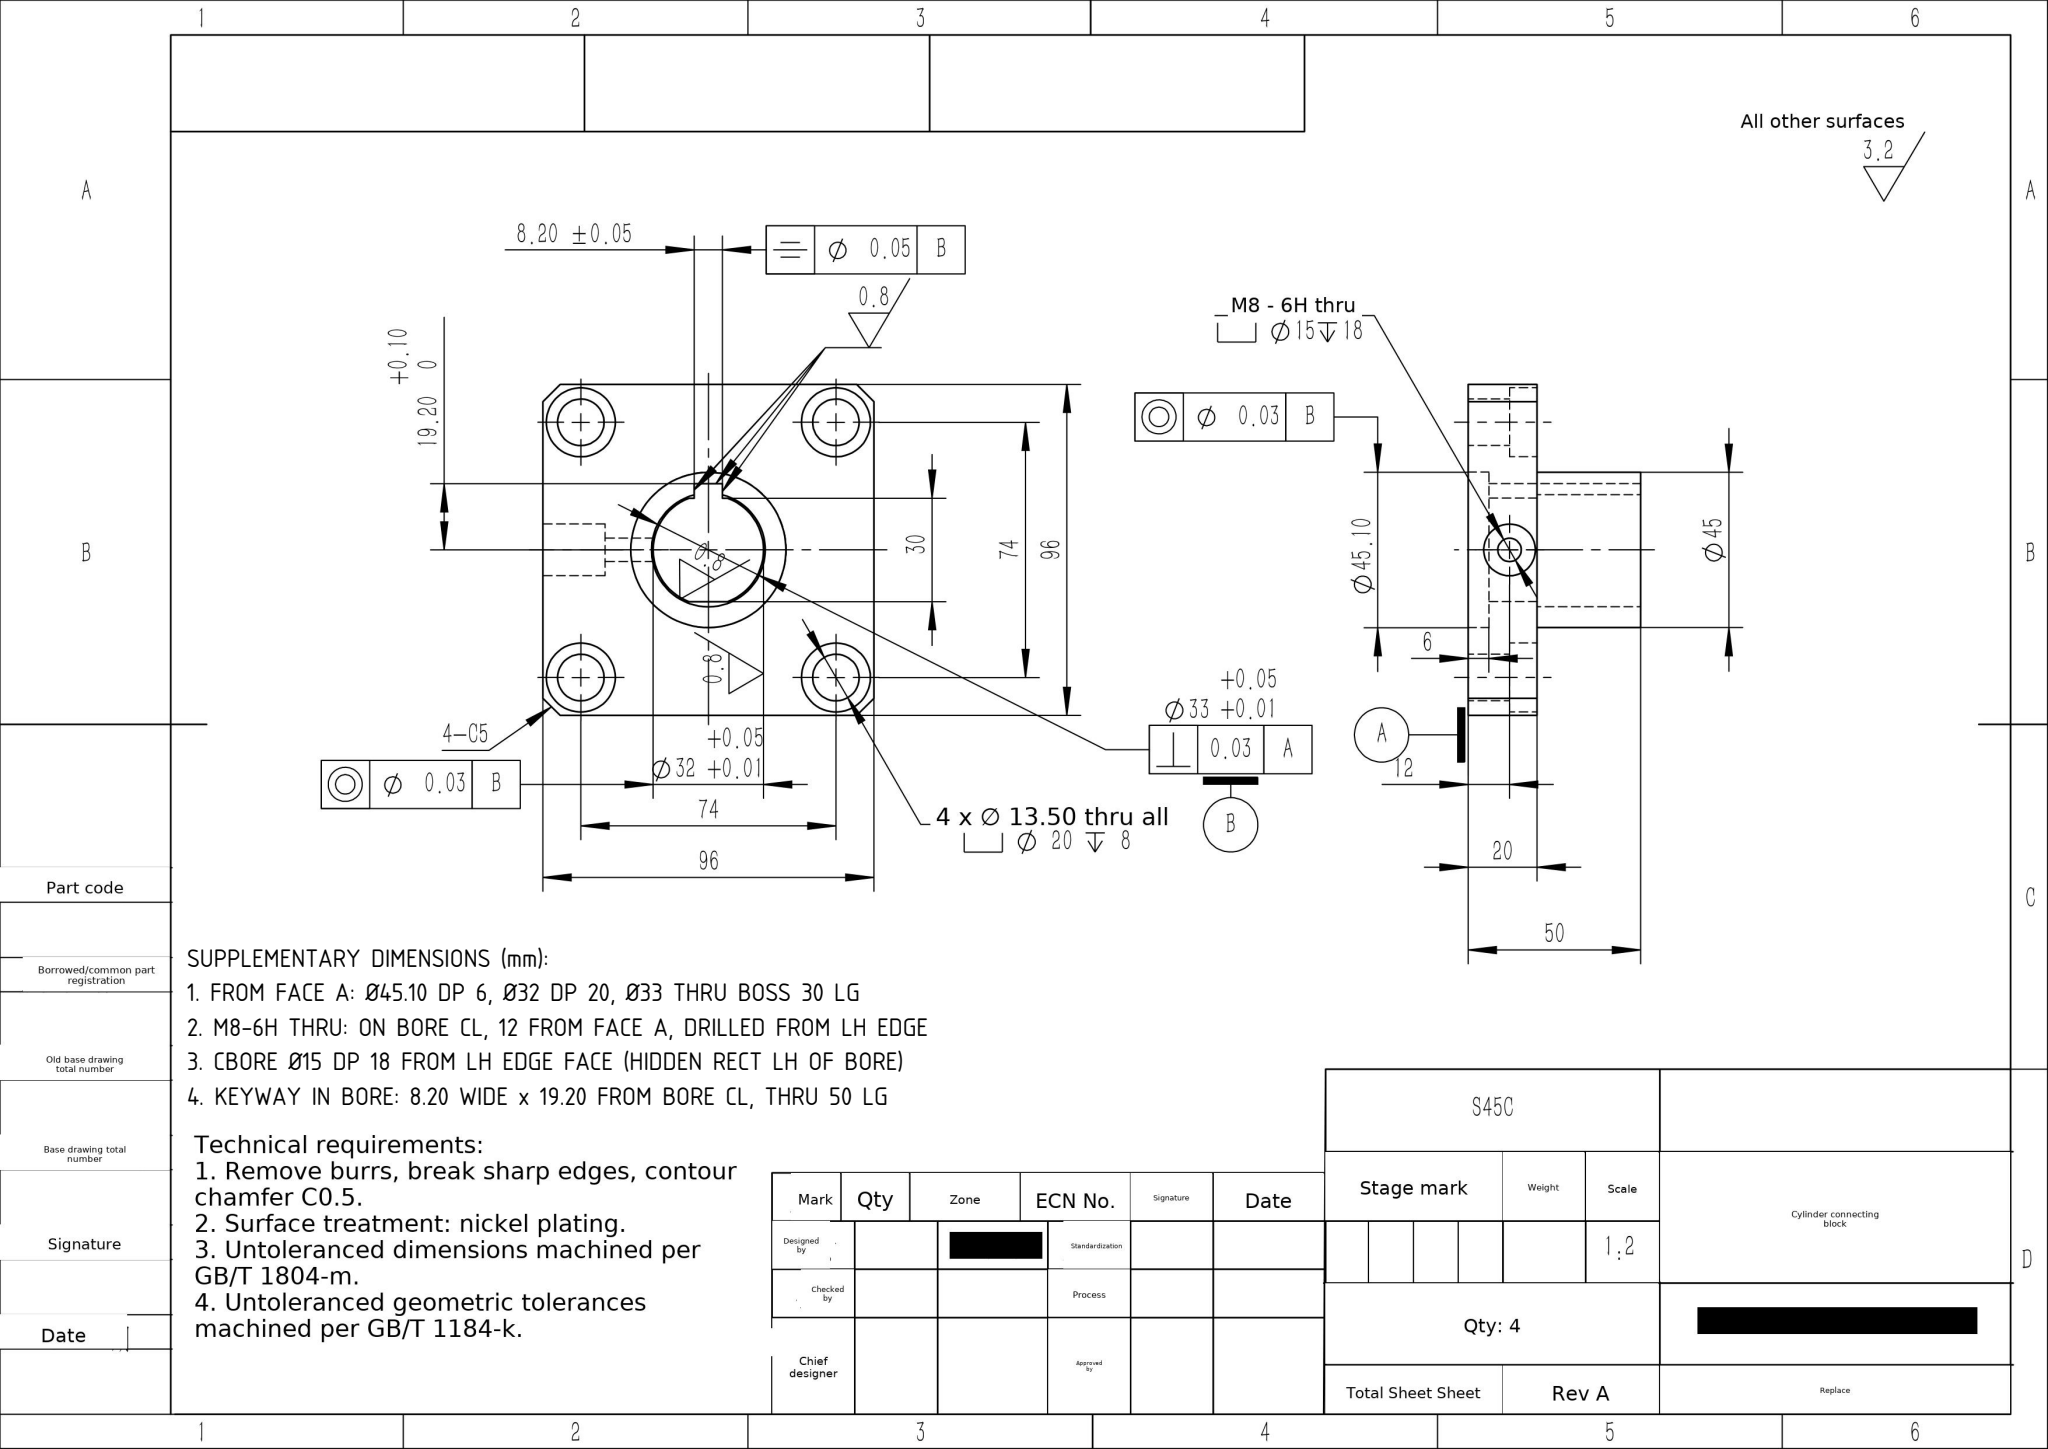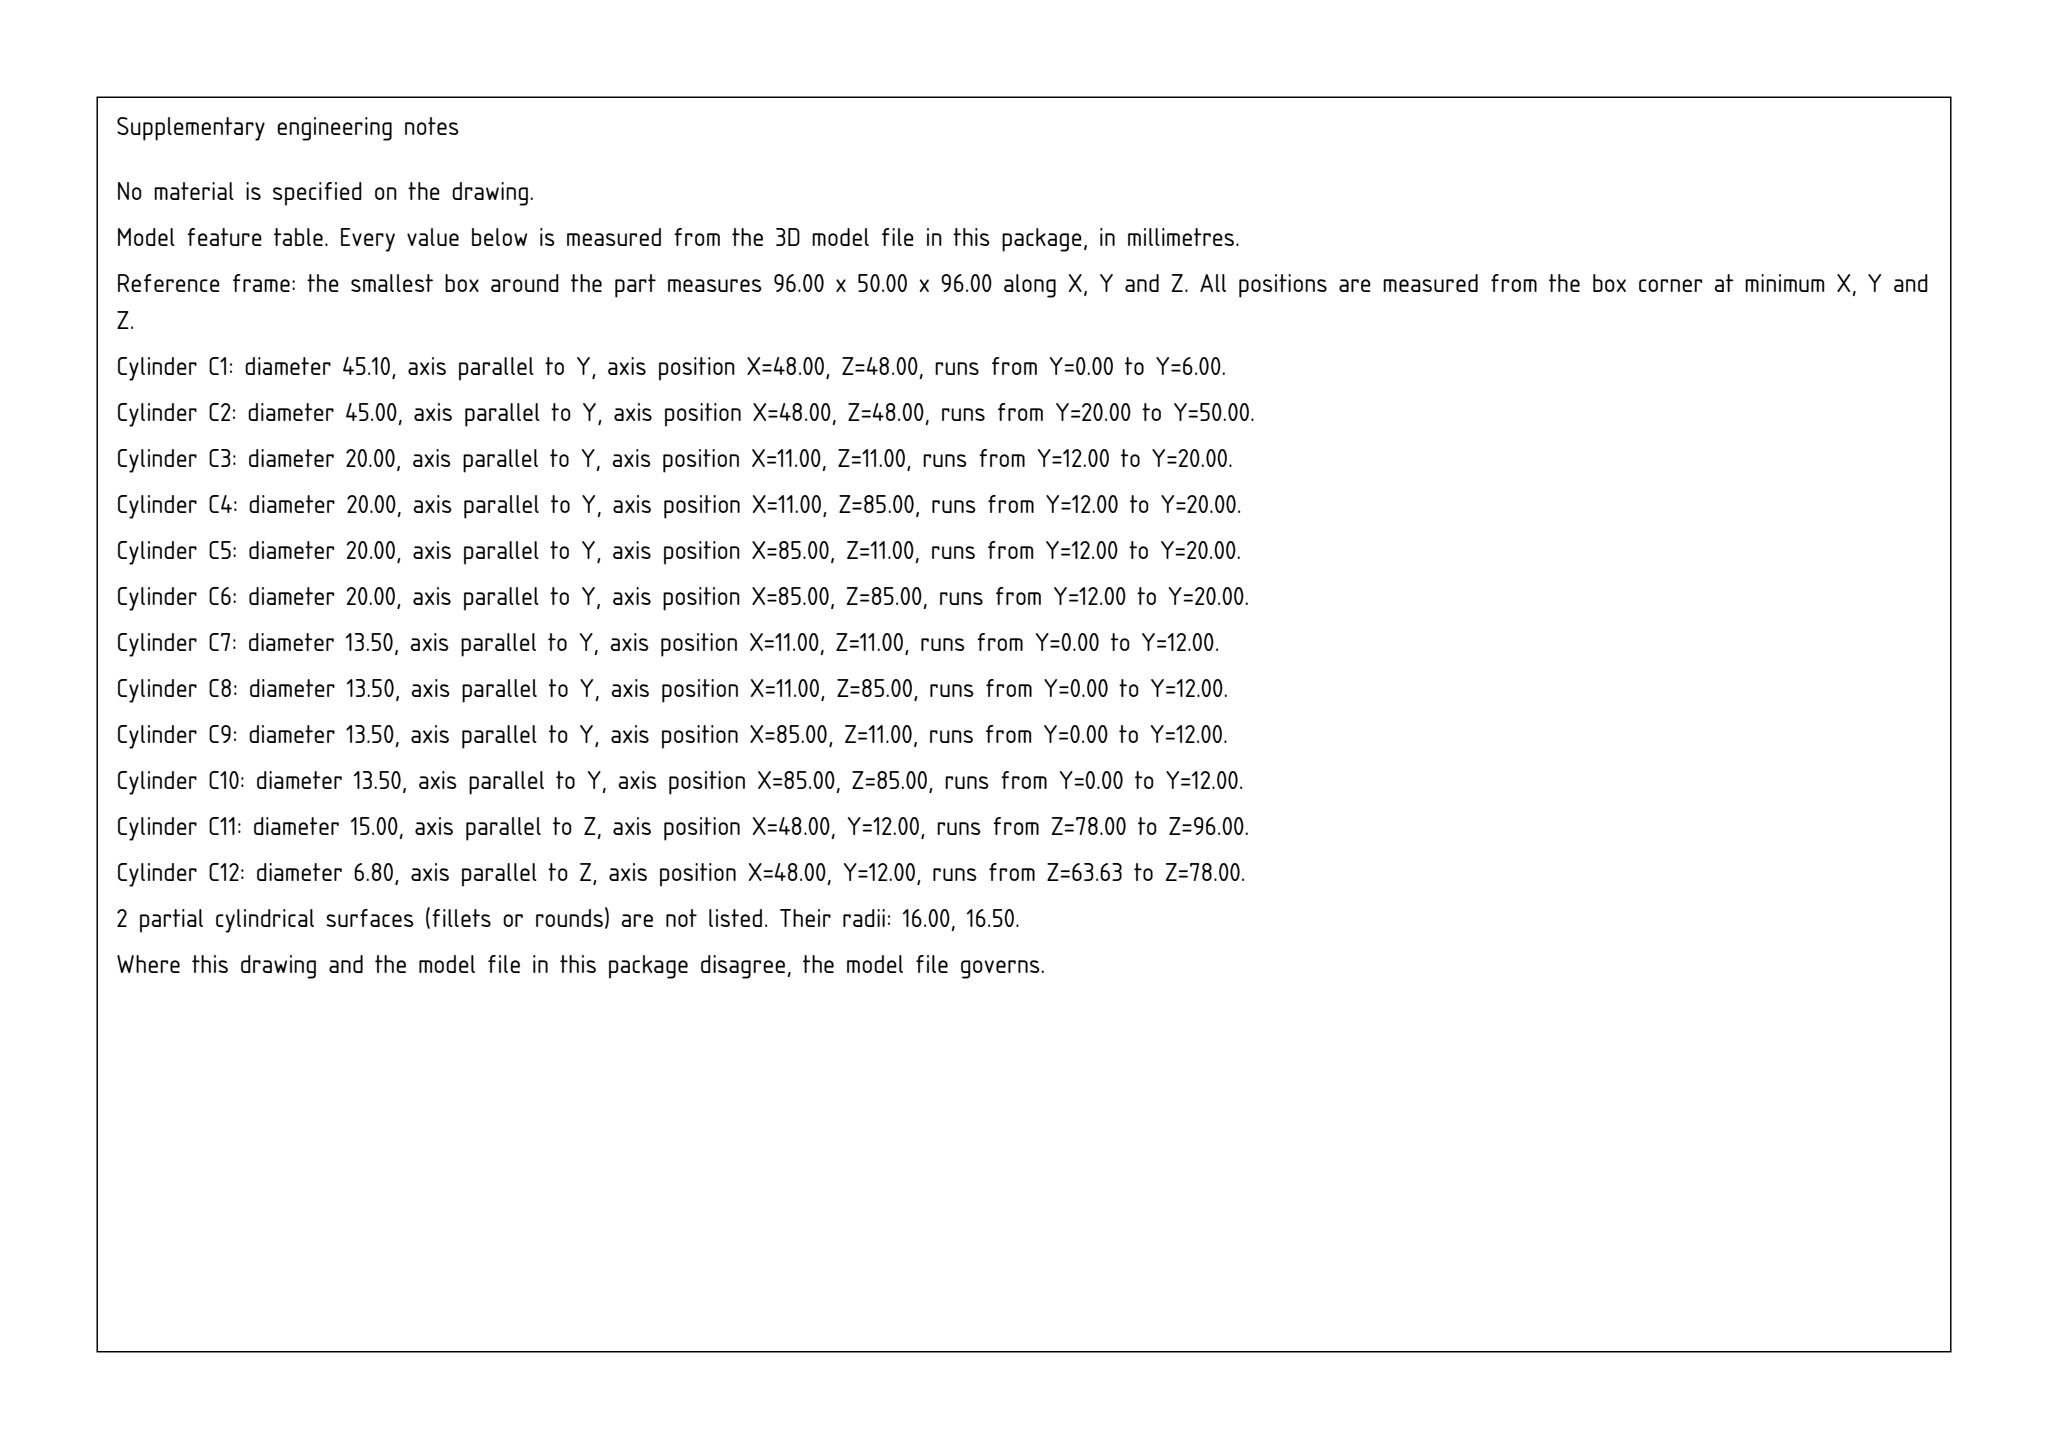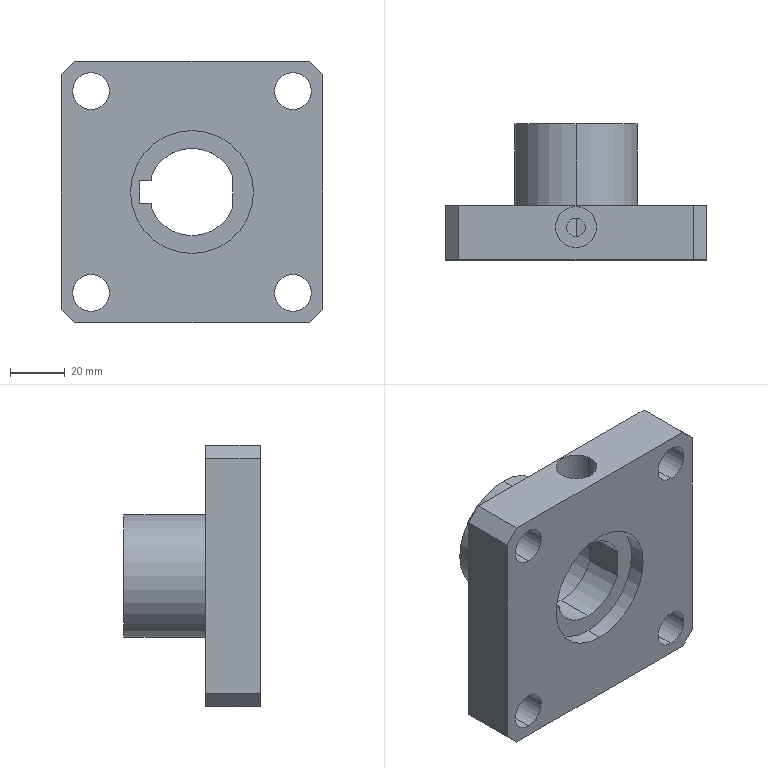Part | SolidWorks | mm | 1 solid | 54 faces | box 96 x 50 x 96 mm | volume 162934 mm3 | cylinder 30 | plane 24 | commonest cylinder face diameters 20 x8 13.5 x8 32 x3 33 x3 15 x2 45.1 x2 45 x2 6.8 x2
build123d program:
from build123d import *

# Parameters (mm, degrees)
SKETCH1_W                                         = 96
SKETCH1_H                                         = 96
BOSS_EXTRUDE1_DEPTH                               = 20
SKETCH2_R                                         = 22.5
BOSS_EXTRUDE2_DEPTH                               = 30
CUT_EXTRUDE1_DEPTH                                = 30
CUT_EXTRUDE2_DEPTH                                = 145.679
SKETCH10_W                                        = 8.572
SKETCH10_H                                        = 8.2
CUT_EXTRUDE3_DEPTH                                = 145.679
SKETCH5_W                                         = 22.55
SKETCH5_H                                         = 6
M8_TAPPED_HOLE1_REACH                             = 202.102
M8_TAPPED_HOLE1_BORE_R                            = 3.4
HOLE_SIZE_ACCORDING_TO_HEXALOBULAR_SO_D           = 13.5
HOLE_SIZE_ACCORDING_TO_HEXALOBULAR_SO_CBORE_D     = 20
HOLE_SIZE_ACCORDING_TO_HEXALOBULAR_SO_CBORE_DEPTH = 8
SKETCH11_R                                        = 7.5
CUT_EXTRUDE4_DEPTH                                = 18
CHAMFER1_SIZE                                     = 5


with BuildPart() as part:
    # Sketch1 → Boss-Extrude1 (new body)
    with BuildSketch(Plane(origin=(0, -127, 0), x_dir=(1, 0, 0), z_dir=(0, 1, 0))):
        with Locations((48, -48)):
            Rectangle(SKETCH1_W, SKETCH1_H)
    extrude(amount=-BOSS_EXTRUDE1_DEPTH)

    # Sketch2 → Boss-Extrude2 (add)
    with BuildSketch(Plane(origin=(0, -127, 0), x_dir=(-1, 0, 0), z_dir=(0, 1, 0))):
        with Locations(Location((-48, 48, 0), (0, 0, 90))):
            Circle(SKETCH2_R)
    extrude(amount=BOSS_EXTRUDE2_DEPTH)

    # Sketch3 → Cut-Extrude1 (cut)
    with BuildSketch(Plane(origin=(0, -97, 0), x_dir=(-1, 0, 0), z_dir=(0, 1, 0))):
        with BuildLine():
            Line((-28.8, 52.1), (-32.018, 52.1))
            ThreePointArc((-32.018, 52.1), (-64.5, 48), (-32.018, 43.9))
            Line((-32.018, 43.9), (-28.8, 43.9))
            Line((-28.8, 43.9), (-28.8, 52.1))
        make_face()
    extrude(amount=-CUT_EXTRUDE1_DEPTH, mode=Mode.SUBTRACT)

    # Sketch4 → Cut-Extrude2 (cut, through all)
    with BuildSketch(Plane.XZ.offset(147)):
        with BuildLine():
            Line((33, 53.568), (33, 42.432))
            ThreePointArc((33, 42.432), (48, 32), (63, 42.432))
            Line((63, 42.432), (63, 53.568))
            ThreePointArc((63, 53.568), (48, 64), (33, 53.568))
        make_face()
    extrude(amount=-CUT_EXTRUDE2_DEPTH, mode=Mode.SUBTRACT)

    # Sketch10 → Cut-Extrude3 (cut, through all)
    with BuildSketch(Plane(origin=(0, -97, 0), x_dir=(1, 0, 0), z_dir=(0, 1, 0))):
        with Locations((33.086, -48)):
            Rectangle(SKETCH10_W, SKETCH10_H)
    extrude(amount=-CUT_EXTRUDE3_DEPTH, mode=Mode.SUBTRACT)

    # Sketch5 → Cut-Revolve1 (revolve, cut)
    with BuildSketch(Plane(origin=(48, 0, 0), x_dir=(0, 0, -1), z_dir=(1, 0, 0))):
        with Locations((-36.725, -144)):
            Rectangle(SKETCH5_W, SKETCH5_H)
    revolve(axis=Axis((48, -141, 48), (0, -1, 0)), mode=Mode.SUBTRACT)

    # M8 Tapped Hole1 bore → M8 Tapped Hole1 (cut, up to next)
    with BuildSketch(Plane.XY.offset(96), mode=Mode.PRIVATE) as m8_tapped_hole1_sk1:
        with Locations((48, -135)):
            Circle(M8_TAPPED_HOLE1_BORE_R)
    m8_tapped_hole1_tool1 = extrude(m8_tapped_hole1_sk1.sketch, amount=-M8_TAPPED_HOLE1_REACH, mode=Mode.PRIVATE) & part.part
    add(m8_tapped_hole1_tool1.solids().sort_by_distance((48, -135, 96))[0], mode=Mode.SUBTRACT)

    # Hole Size _ According to_ Hexalobular So (through all)
    with Locations(Plane(origin=(0, -127, 0), x_dir=(1, 0, 0), z_dir=(0, 1, 0))):
        with Locations((11, -11), (85, -11), (85, -85), (11, -85)):
            CounterBoreHole(HOLE_SIZE_ACCORDING_TO_HEXALOBULAR_SO_D / 2, HOLE_SIZE_ACCORDING_TO_HEXALOBULAR_SO_CBORE_D / 2, HOLE_SIZE_ACCORDING_TO_HEXALOBULAR_SO_CBORE_DEPTH)

    # Sketch11 → Cut-Extrude4 (cut)
    with BuildSketch(Plane.XY.offset(96)):
        with Locations((48, -135)):
            Circle(SKETCH11_R)
    extrude(amount=-CUT_EXTRUDE4_DEPTH, mode=Mode.SUBTRACT)

    # Chamfer1
    chamfer1_edges = [part.edges().sort_by_distance(p)[0] for p in [
        (96, -137, 96),
        (0, -137, 96),
        (0, -137, 0),
        (96, -137, 0),
    ]]
    chamfer(chamfer1_edges, length=CHAMFER1_SIZE)


solid = part.part